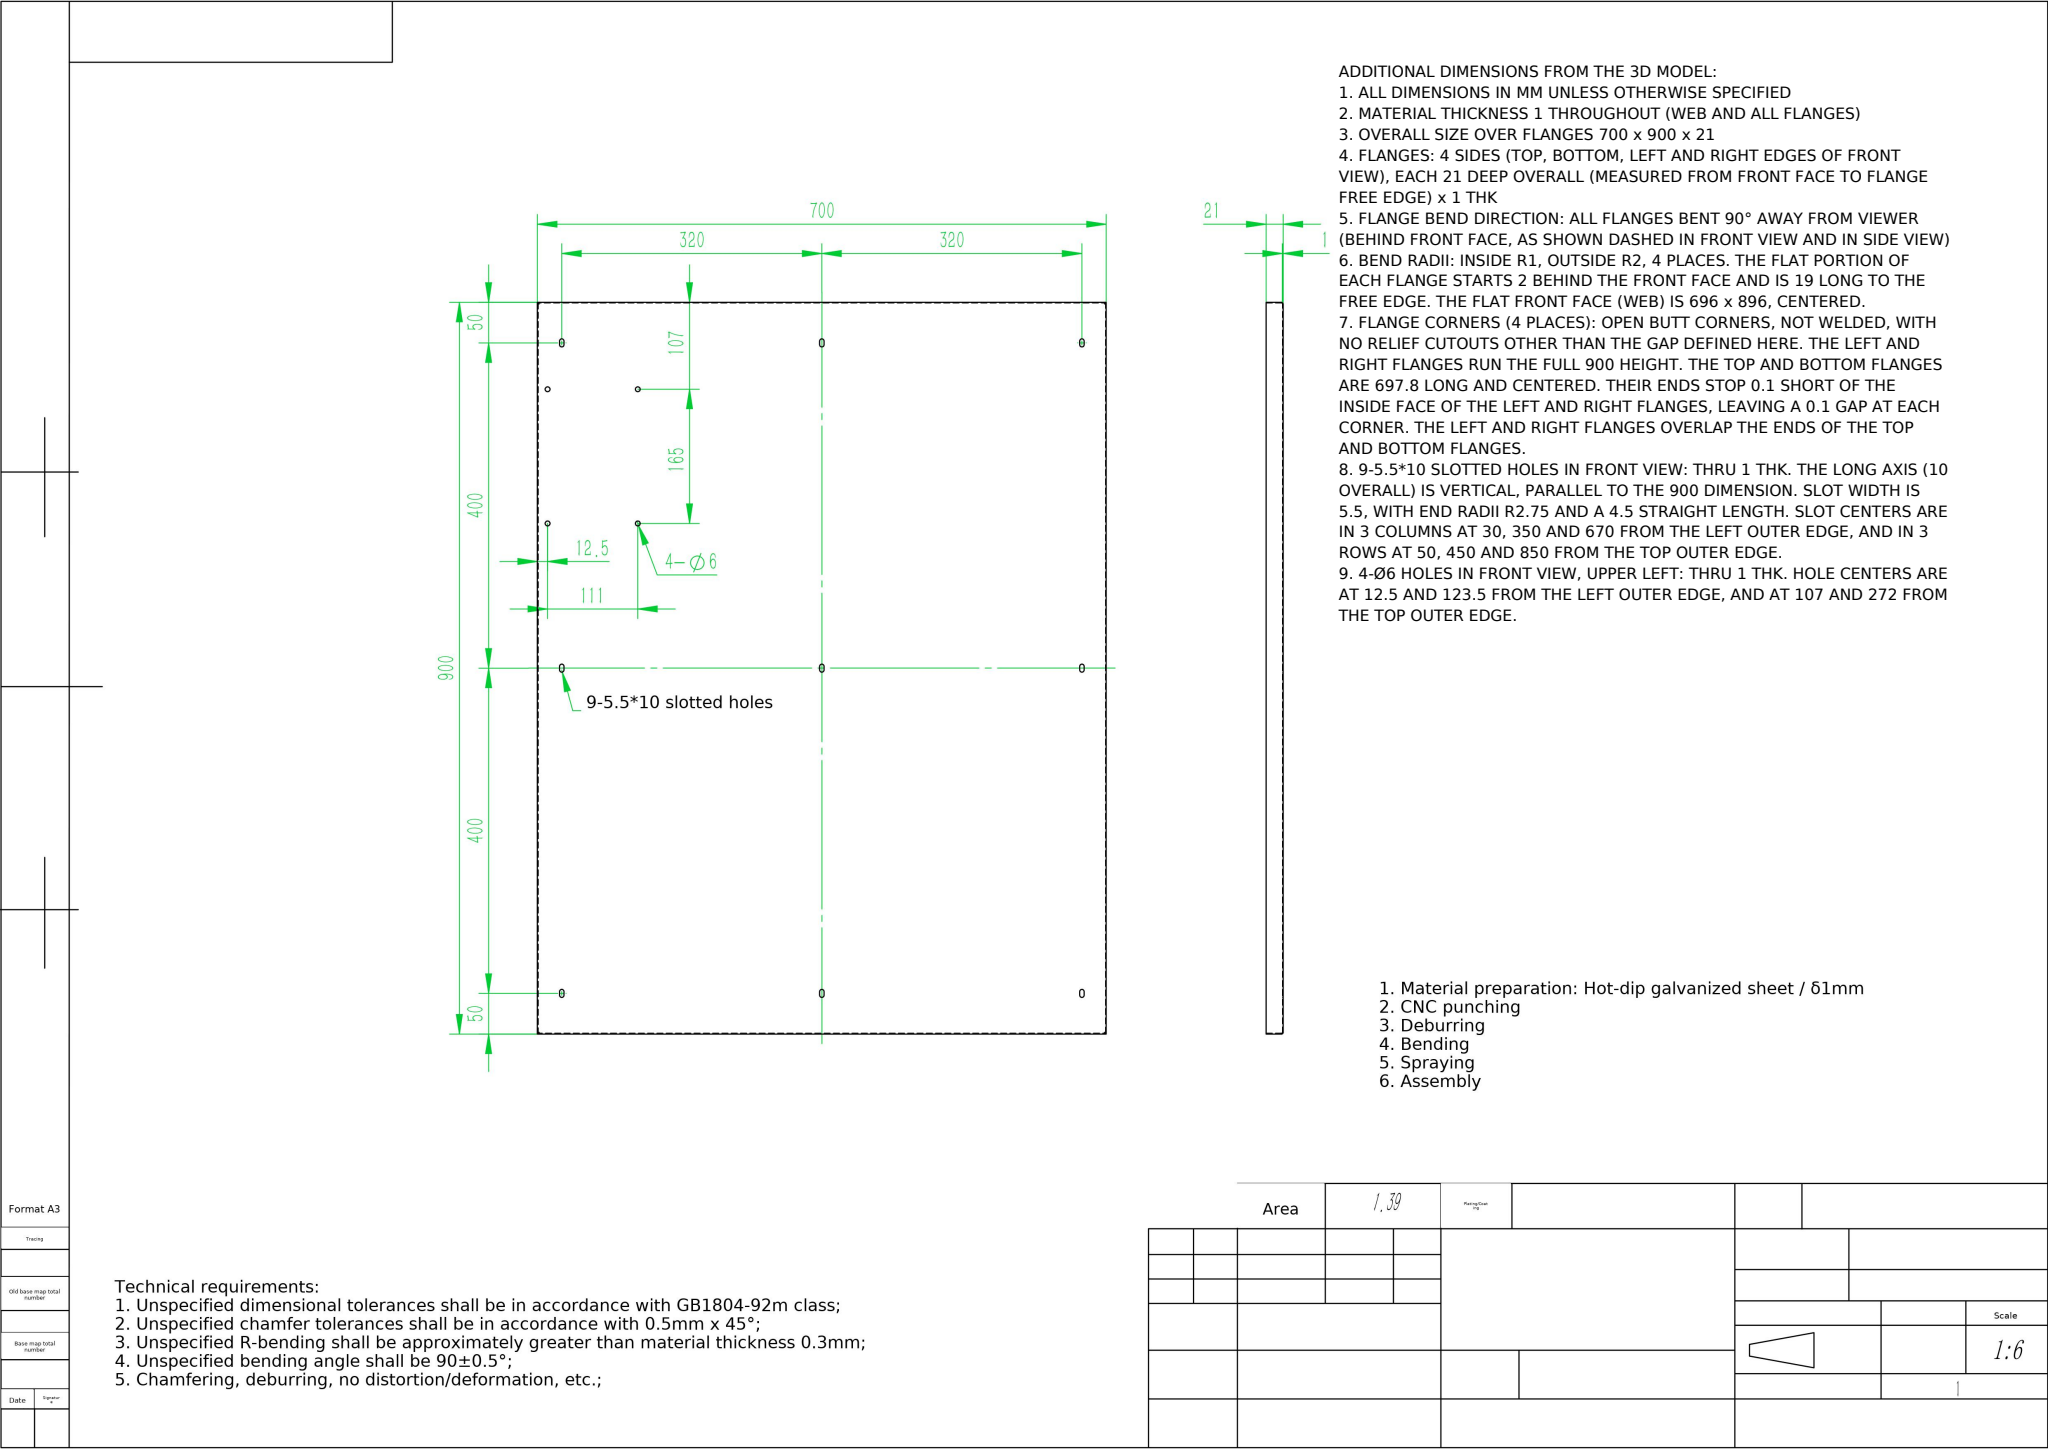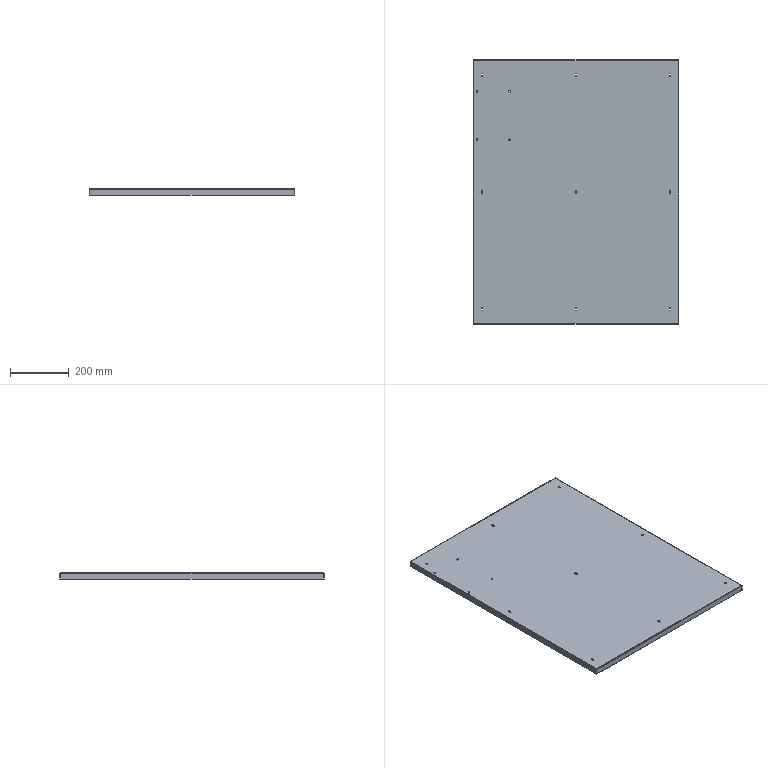Part | NX | mm | 1 solid | 82 faces | box 700 x 900 x 21 mm | volume 691299 mm3 | plane 40 | cylinder 34 | spline 8 | commonest cylinder face diameters 5.5 x18 6 x8 2 x4 4 x4